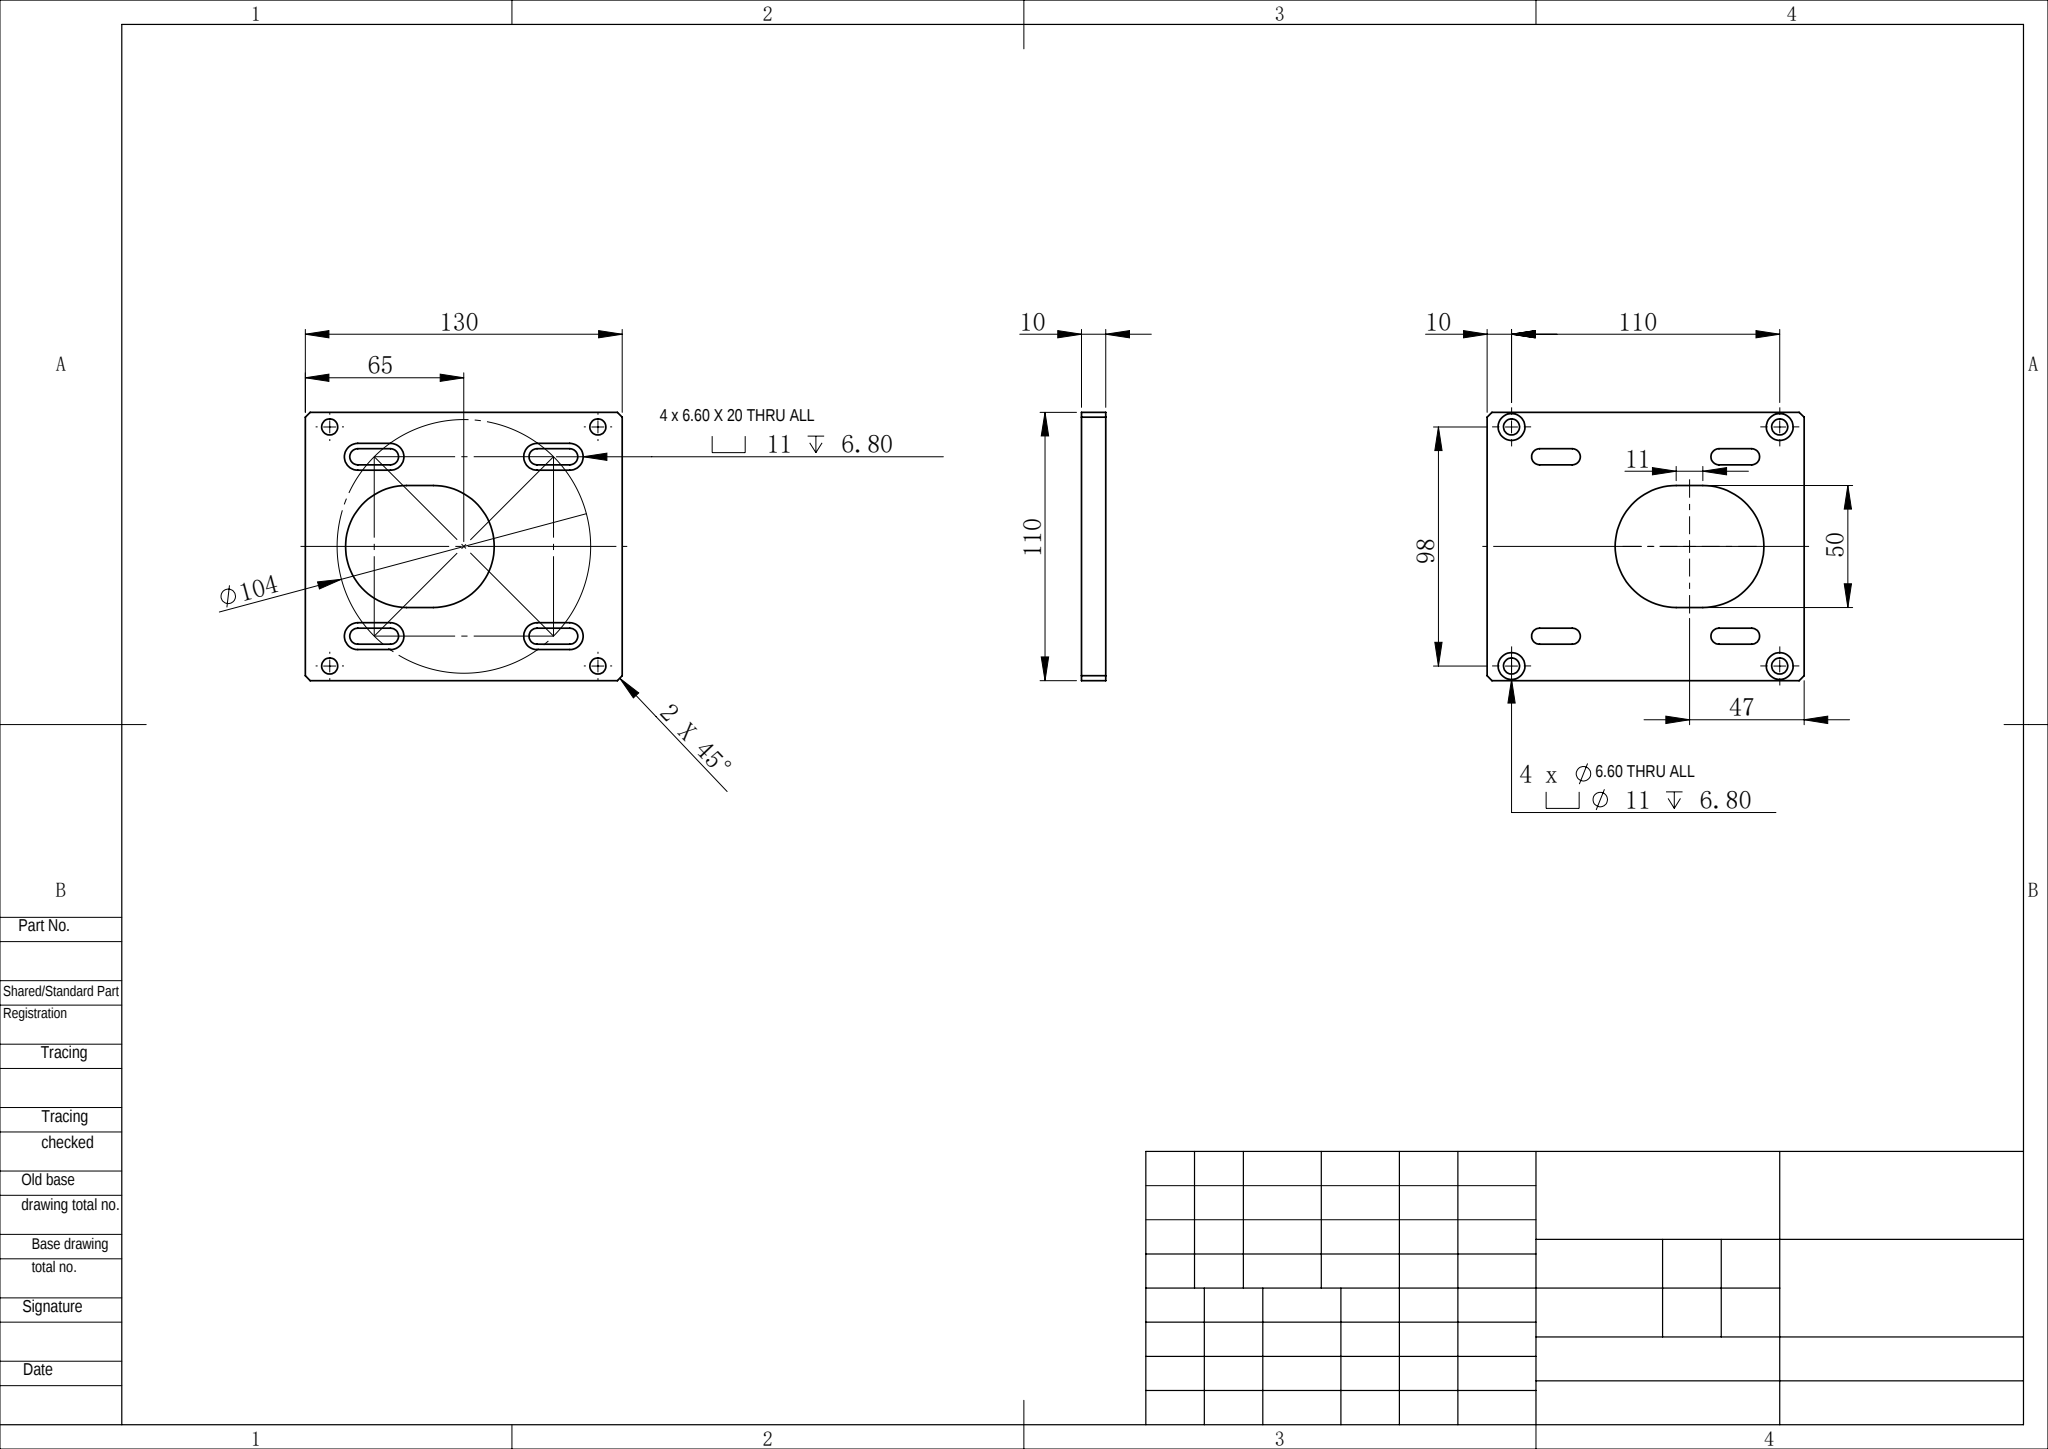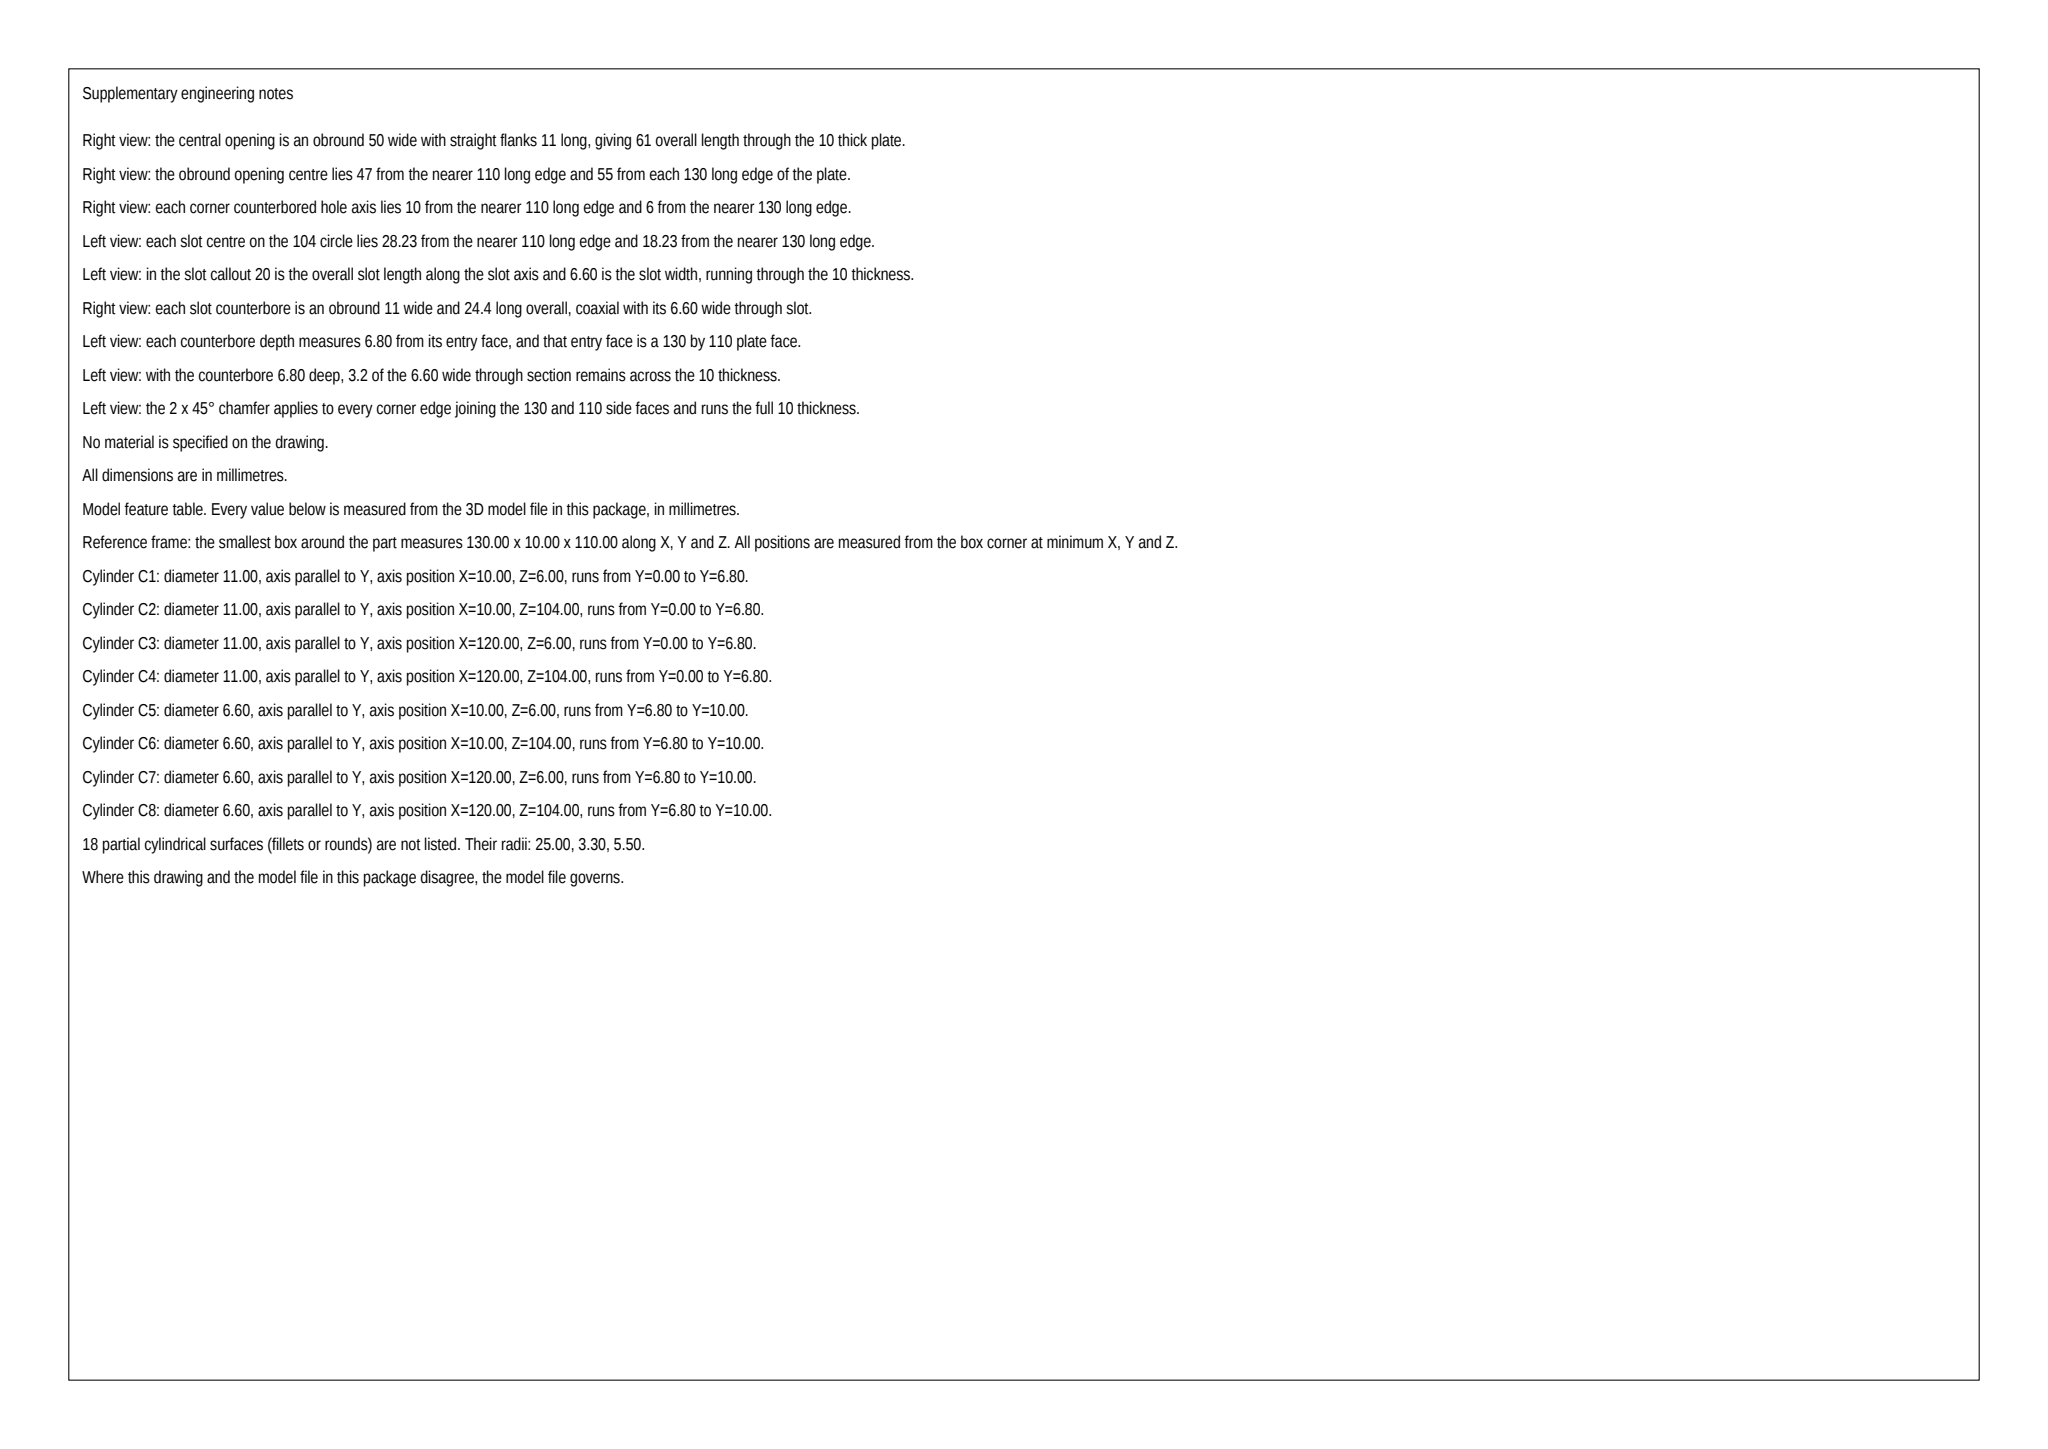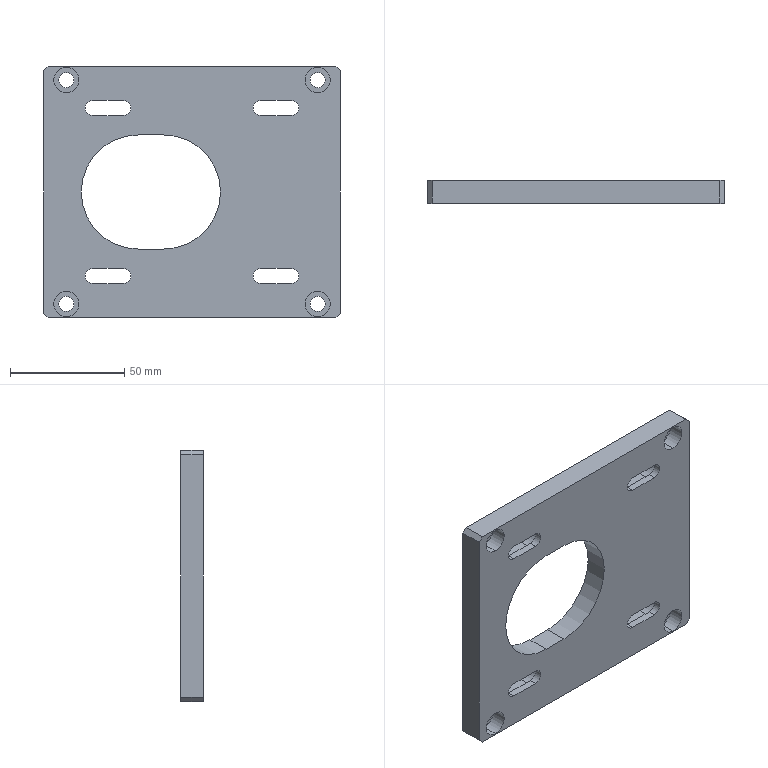Part | SolidWorks | mm | 1 solid | 70 faces | box 130 x 10 x 110 mm | volume 106598 mm3 | plane 36 | cylinder 34 | commonest cylinder face diameters 11 x16 6.6 x16 50 x2